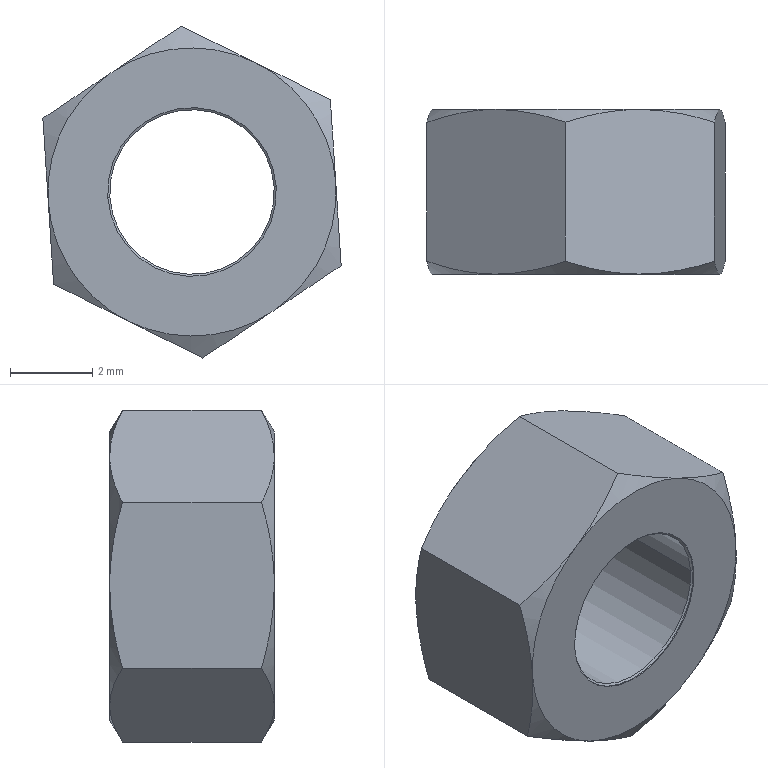Component | SolidWorks | hex nut style 2_am_pkg-24 | 1 solid | 28 faces | box 7.25 x 4 x 8.07 mm | volume 119 mm3 | cone 16 | plane 8 | cylinder 4 | commonest cylinder face diameters 4.1 x2 4 x2
STEP:
#1=COLOUR_RGB('',0.7922,0.8196,0.9333);
#2=FILL_AREA_STYLE_COLOUR('',#1);
#3=FILL_AREA_STYLE('',(#2));
#4=SURFACE_STYLE_FILL_AREA(#3);
#5=SURFACE_SIDE_STYLE('',(#4));
#6=SURFACE_STYLE_USAGE(.BOTH.,#5);
#7=PRESENTATION_STYLE_ASSIGNMENT((#6));
#8=CARTESIAN_POINT('',(-3.26,1.437,3.346));
#9=VERTEX_POINT('',#8);
#10=CARTESIAN_POINT('',(-3.421,1.437,3.335));
#11=VERTEX_POINT('',#10);
#12=CARTESIAN_POINT('',(-3.341,1.437,3.341));
#13=DIRECTION('',(-0.,1.,0.));
#14=DIRECTION('',(0.9979,0.,0.06475));
#15=AXIS2_PLACEMENT_3D('',#12,#13,#14);
#16=CIRCLE('',#15,0.08071);
#17=EDGE_CURVE('',#9,#11,#16,.T.);
#18=ORIENTED_EDGE('',*,*,#17,.F.);
#19=CARTESIAN_POINT('',(-3.26,1.438,3.346));
#20=VERTEX_POINT('',#19);
#21=CARTESIAN_POINT('',(-3.26,0.6088,3.346));
#22=DIRECTION('',(-0.,1.,0.));
#23=VECTOR('',#22,39.37);
#24=LINE('',#21,#23);
#25=EDGE_CURVE('',#9,#20,#24,.T.);
#26=ORIENTED_EDGE('',*,*,#25,.T.);
#27=CARTESIAN_POINT('',(-3.421,1.438,3.335));
#28=VERTEX_POINT('',#27);
#29=CARTESIAN_POINT('',(-3.341,1.438,3.341));
#30=DIRECTION('',(-0.,1.,0.));
#31=DIRECTION('',(-0.9979,0.,-0.06475));
#32=AXIS2_PLACEMENT_3D('',#29,#30,#31);
#33=CIRCLE('',#32,0.08071);
#34=EDGE_CURVE('',#20,#28,#33,.T.);
#35=ORIENTED_EDGE('',*,*,#34,.T.);
#36=CARTESIAN_POINT('',(-3.421,0.6088,3.335));
#37=DIRECTION('',(-0.,1.,0.));
#38=VECTOR('',#37,39.37);
#39=LINE('',#36,#38);
#40=EDGE_CURVE('',#11,#28,#39,.T.);
#41=ORIENTED_EDGE('',*,*,#40,.F.);
#42=EDGE_LOOP('',(#18,#26,#35,#41));
#43=FACE_OUTER_BOUND('',#42,.T.);
#44=CARTESIAN_POINT('',(-3.341,0.6088,3.341));
#45=DIRECTION('',(-0.,1.,0.));
#46=DIRECTION('',(-0.9979,0.,-0.06475));
#47=AXIS2_PLACEMENT_3D('',#44,#45,#46);
#48=CYLINDRICAL_SURFACE('',#47,0.08071);
#49=ADVANCED_FACE('',(#43),#48,.F.);
#50=CARTESIAN_POINT('',(-3.262,1.439,3.346));
#51=VERTEX_POINT('',#50);
#52=CARTESIAN_POINT('',(-3.419,1.439,3.336));
#53=VERTEX_POINT('',#52);
#54=CARTESIAN_POINT('',(-3.341,1.439,3.341));
#55=DIRECTION('',(-0.,1.,0.));
#56=DIRECTION('',(0.9979,0.,0.06475));
#57=AXIS2_PLACEMENT_3D('',#54,#55,#56);
#58=CIRCLE('',#57,0.07874);
#59=EDGE_CURVE('',#51,#53,#58,.T.);
#60=ORIENTED_EDGE('',*,*,#59,.T.);
#61=CARTESIAN_POINT('',(-3.421,1.438,3.335));
#62=DIRECTION('',(-0.8174,-0.5736,-0.05304));
#63=VECTOR('',#62,39.37);
#64=LINE('',#61,#63);
#65=EDGE_CURVE('',#53,#28,#64,.T.);
#66=ORIENTED_EDGE('',*,*,#65,.T.);
#67=ORIENTED_EDGE('',*,*,#34,.F.);
#68=CARTESIAN_POINT('',(-3.26,1.438,3.346));
#69=DIRECTION('',(0.8174,-0.5736,0.05304));
#70=VECTOR('',#69,39.37);
#71=LINE('',#68,#70);
#72=EDGE_CURVE('',#51,#20,#71,.T.);
#73=ORIENTED_EDGE('',*,*,#72,.F.);
#74=EDGE_LOOP('',(#60,#66,#67,#73));
#75=FACE_OUTER_BOUND('',#74,.T.);
#76=CARTESIAN_POINT('',(-3.341,1.438,3.341));
#77=DIRECTION('',(0.,-1.,-0.));
#78=DIRECTION('',(0.9979,0.,0.06475));
#79=AXIS2_PLACEMENT_3D('',#76,#77,#78);
#80=CONICAL_SURFACE('',#79,0.08071,0.9599);
#81=ADVANCED_FACE('',(#75),#80,.F.);
#82=CARTESIAN_POINT('',(-3.419,1.593,3.336));
#83=VERTEX_POINT('',#82);
#84=CARTESIAN_POINT('',(-3.262,1.593,3.346));
#85=VERTEX_POINT('',#84);
#86=CARTESIAN_POINT('',(-3.341,1.593,3.341));
#87=DIRECTION('',(0.,-1.,-0.));
#88=DIRECTION('',(-0.9979,0.,-0.06475));
#89=AXIS2_PLACEMENT_3D('',#86,#87,#88);
#90=CIRCLE('',#89,0.07874);
#91=EDGE_CURVE('',#83,#85,#90,.T.);
#92=ORIENTED_EDGE('',*,*,#91,.T.);
#93=CARTESIAN_POINT('',(-3.26,1.594,3.346));
#94=VERTEX_POINT('',#93);
#95=CARTESIAN_POINT('',(-3.262,1.593,3.346));
#96=DIRECTION('',(0.8174,0.5736,0.05304));
#97=VECTOR('',#96,39.37);
#98=LINE('',#95,#97);
#99=EDGE_CURVE('',#85,#94,#98,.T.);
#100=ORIENTED_EDGE('',*,*,#99,.T.);
#101=CARTESIAN_POINT('',(-3.421,1.594,3.335));
#102=VERTEX_POINT('',#101);
#103=CARTESIAN_POINT('',(-3.341,1.594,3.341));
#104=DIRECTION('',(-0.,1.,0.));
#105=DIRECTION('',(-0.9979,0.,-0.06475));
#106=AXIS2_PLACEMENT_3D('',#103,#104,#105);
#107=CIRCLE('',#106,0.08071);
#108=EDGE_CURVE('',#94,#102,#107,.T.);
#109=ORIENTED_EDGE('',*,*,#108,.T.);
#110=CARTESIAN_POINT('',(-3.419,1.593,3.336));
#111=DIRECTION('',(-0.8174,0.5736,-0.05304));
#112=VECTOR('',#111,39.37);
#113=LINE('',#110,#112);
#114=EDGE_CURVE('',#83,#102,#113,.T.);
#115=ORIENTED_EDGE('',*,*,#114,.F.);
#116=EDGE_LOOP('',(#92,#100,#109,#115));
#117=FACE_OUTER_BOUND('',#116,.T.);
#118=CARTESIAN_POINT('',(-3.341,1.593,3.341));
#119=DIRECTION('',(-0.,1.,0.));
#120=DIRECTION('',(-0.9979,0.,-0.06475));
#121=AXIS2_PLACEMENT_3D('',#118,#119,#120);
#122=CONICAL_SURFACE('',#121,0.07854,0.9599);
#123=ADVANCED_FACE('',(#117),#122,.F.);
#124=ORIENTED_EDGE('',*,*,#59,.F.);
#125=CARTESIAN_POINT('',(-3.262,1.437,3.346));
#126=DIRECTION('',(-0.,1.,0.));
#127=VECTOR('',#126,39.37);
#128=LINE('',#125,#127);
#129=EDGE_CURVE('',#51,#85,#128,.T.);
#130=ORIENTED_EDGE('',*,*,#129,.T.);
#131=ORIENTED_EDGE('',*,*,#91,.F.);
#132=CARTESIAN_POINT('',(-3.419,1.437,3.336));
#133=DIRECTION('',(-0.,1.,0.));
#134=VECTOR('',#133,39.37);
#135=LINE('',#132,#134);
#136=EDGE_CURVE('',#53,#83,#135,.T.);
#137=ORIENTED_EDGE('',*,*,#136,.F.);
#138=EDGE_LOOP('',(#124,#130,#131,#137));
#139=FACE_OUTER_BOUND('',#138,.T.);
#140=CARTESIAN_POINT('',(-3.341,1.437,3.341));
#141=DIRECTION('',(-0.,1.,0.));
#142=DIRECTION('',(-0.9979,0.,-0.06475));
#143=AXIS2_PLACEMENT_3D('',#140,#141,#142);
#144=CYLINDRICAL_SURFACE('',#143,0.07874);
#145=ADVANCED_FACE('',(#139),#144,.F.);
#146=ORIENTED_EDGE('',*,*,#129,.F.);
#147=CARTESIAN_POINT('',(-3.341,1.439,3.341));
#148=DIRECTION('',(-0.,1.,0.));
#149=DIRECTION('',(0.9979,0.,0.06475));
#150=AXIS2_PLACEMENT_3D('',#147,#148,#149);
#151=CIRCLE('',#150,0.07874);
#152=EDGE_CURVE('',#53,#51,#151,.T.);
#153=ORIENTED_EDGE('',*,*,#152,.F.);
#154=ORIENTED_EDGE('',*,*,#136,.T.);
#155=CARTESIAN_POINT('',(-3.341,1.593,3.341));
#156=DIRECTION('',(0.,-1.,-0.));
#157=DIRECTION('',(-0.9979,0.,-0.06475));
#158=AXIS2_PLACEMENT_3D('',#155,#156,#157);
#159=CIRCLE('',#158,0.07874);
#160=EDGE_CURVE('',#85,#83,#159,.T.);
#161=ORIENTED_EDGE('',*,*,#160,.F.);
#162=EDGE_LOOP('',(#146,#153,#154,#161));
#163=FACE_OUTER_BOUND('',#162,.T.);
#164=CARTESIAN_POINT('',(-3.341,1.437,3.341));
#165=DIRECTION('',(-0.,1.,0.));
#166=DIRECTION('',(-0.9979,0.,-0.06475));
#167=AXIS2_PLACEMENT_3D('',#164,#165,#166);
#168=CYLINDRICAL_SURFACE('',#167,0.07874);
#169=ADVANCED_FACE('',(#163),#168,.F.);
#170=CARTESIAN_POINT('',(-3.208,1.449,3.429));
#171=VERTEX_POINT('',#170);
#172=CARTESIAN_POINT('',(-3.208,1.582,3.429));
#173=VERTEX_POINT('',#172);
#174=CARTESIAN_POINT('',(-3.208,1.437,3.429));
#175=DIRECTION('',(-0.,1.,0.));
#176=VECTOR('',#175,39.37);
#177=LINE('',#174,#176);
#178=EDGE_CURVE('',#171,#173,#177,.T.);
#179=ORIENTED_EDGE('',*,*,#178,.T.);
#180=CARTESIAN_POINT('',(-3.28,1.594,3.464));
#181=VERTEX_POINT('',#180);
#182=CARTESIAN_POINT('',(-3.208,1.582,3.429));
#183=CARTESIAN_POINT('',(-3.232,1.59,3.441));
#184=CARTESIAN_POINT('',(-3.255,1.594,3.452));
#185=CARTESIAN_POINT('',(-3.28,1.594,3.464));
#186=B_SPLINE_CURVE_WITH_KNOTS('',3,(#182,#183,#184,#185),.UNSPECIFIED.,.F.,.F.,(4,4),(0.00000024,0.002045),.UNSPECIFIED.);
#187=EDGE_CURVE('',#173,#181,#186,.T.);
#188=ORIENTED_EDGE('',*,*,#187,.T.);
#189=CARTESIAN_POINT('',(-3.351,1.582,3.499));
#190=VERTEX_POINT('',#189);
#191=CARTESIAN_POINT('',(-3.28,1.594,3.464));
#192=CARTESIAN_POINT('',(-3.292,1.594,3.47));
#193=CARTESIAN_POINT('',(-3.304,1.593,3.476));
#194=CARTESIAN_POINT('',(-3.328,1.589,3.488));
#195=CARTESIAN_POINT('',(-3.339,1.586,3.494));
#196=CARTESIAN_POINT('',(-3.351,1.582,3.499));
#197=B_SPLINE_CURVE_WITH_KNOTS('',3,(#191,#192,#193,#194,#195,#196),.UNSPECIFIED.,.F.,.F.,(4,2,4),(0.002045,0.003063,0.004082),.UNSPECIFIED.);
#198=EDGE_CURVE('',#181,#190,#197,.T.);
#199=ORIENTED_EDGE('',*,*,#198,.T.);
#200=CARTESIAN_POINT('',(-3.351,1.449,3.499));
#201=VERTEX_POINT('',#200);
#202=CARTESIAN_POINT('',(-3.351,1.437,3.499));
#203=DIRECTION('',(-0.,1.,0.));
#204=VECTOR('',#203,39.37);
#205=LINE('',#202,#204);
#206=EDGE_CURVE('',#201,#190,#205,.T.);
#207=ORIENTED_EDGE('',*,*,#206,.F.);
#208=CARTESIAN_POINT('',(-3.28,1.437,3.464));
#209=VERTEX_POINT('',#208);
#210=CARTESIAN_POINT('',(-3.28,1.437,3.464));
#211=CARTESIAN_POINT('',(-3.292,1.437,3.47));
#212=CARTESIAN_POINT('',(-3.304,1.438,3.476));
#213=CARTESIAN_POINT('',(-3.328,1.442,3.488));
#214=CARTESIAN_POINT('',(-3.339,1.446,3.494));
#215=CARTESIAN_POINT('',(-3.351,1.449,3.499));
#216=B_SPLINE_CURVE_WITH_KNOTS('',3,(#210,#211,#212,#213,#214,#215),.UNSPECIFIED.,.F.,.F.,(4,2,4),(0.002045,0.003063,0.004082),.UNSPECIFIED.);
#217=EDGE_CURVE('',#209,#201,#216,.T.);
#218=ORIENTED_EDGE('',*,*,#217,.F.);
#219=CARTESIAN_POINT('',(-3.208,1.449,3.429));
#220=CARTESIAN_POINT('',(-3.232,1.442,3.441));
#221=CARTESIAN_POINT('',(-3.255,1.437,3.452));
#222=CARTESIAN_POINT('',(-3.28,1.437,3.464));
#223=B_SPLINE_CURVE_WITH_KNOTS('',3,(#219,#220,#221,#222),.UNSPECIFIED.,.F.,.F.,(4,4),(0.00000024,0.002045),.UNSPECIFIED.);
#224=EDGE_CURVE('',#171,#209,#223,.T.);
#225=ORIENTED_EDGE('',*,*,#224,.F.);
#226=EDGE_LOOP('',(#179,#188,#199,#207,#218,#225));
#227=FACE_OUTER_BOUND('',#226,.T.);
#228=CARTESIAN_POINT('',(-3.351,1.437,3.499));
#229=DIRECTION('',(0.4429,0.,0.8966));
#230=DIRECTION('',(0.8966,0.,-0.4429));
#231=AXIS2_PLACEMENT_3D('',#228,#229,#230);
#232=PLANE('',#231);
#233=ADVANCED_FACE('',(#227),#232,.T.);
#234=ORIENTED_EDGE('',*,*,#206,.T.);
#235=CARTESIAN_POINT('',(-3.417,1.594,3.455));
#236=VERTEX_POINT('',#235);
#237=CARTESIAN_POINT('',(-3.351,1.582,3.499));
#238=CARTESIAN_POINT('',(-3.373,1.59,3.485));
#239=CARTESIAN_POINT('',(-3.395,1.594,3.47));
#240=CARTESIAN_POINT('',(-3.417,1.594,3.455));
#241=B_SPLINE_CURVE_WITH_KNOTS('',3,(#237,#238,#239,#240),.UNSPECIFIED.,.F.,.F.,(4,4),(0.00000024,0.002045),.UNSPECIFIED.);
#242=EDGE_CURVE('',#190,#236,#241,.T.);
#243=ORIENTED_EDGE('',*,*,#242,.T.);
#244=CARTESIAN_POINT('',(-3.483,1.582,3.411));
#245=VERTEX_POINT('',#244);
#246=CARTESIAN_POINT('',(-3.417,1.594,3.455));
#247=CARTESIAN_POINT('',(-3.428,1.594,3.448));
#248=CARTESIAN_POINT('',(-3.44,1.593,3.44));
#249=CARTESIAN_POINT('',(-3.462,1.589,3.426));
#250=CARTESIAN_POINT('',(-3.473,1.586,3.418));
#251=CARTESIAN_POINT('',(-3.483,1.582,3.411));
#252=B_SPLINE_CURVE_WITH_KNOTS('',3,(#246,#247,#248,#249,#250,#251),.UNSPECIFIED.,.F.,.F.,(4,2,4),(0.002045,0.003063,0.004082),.UNSPECIFIED.);
#253=EDGE_CURVE('',#236,#245,#252,.T.);
#254=ORIENTED_EDGE('',*,*,#253,.T.);
#255=CARTESIAN_POINT('',(-3.483,1.449,3.411));
#256=VERTEX_POINT('',#255);
#257=CARTESIAN_POINT('',(-3.483,1.437,3.411));
#258=DIRECTION('',(-0.,1.,0.));
#259=VECTOR('',#258,39.37);
#260=LINE('',#257,#259);
#261=EDGE_CURVE('',#256,#245,#260,.T.);
#262=ORIENTED_EDGE('',*,*,#261,.F.);
#263=CARTESIAN_POINT('',(-3.417,1.437,3.455));
#264=VERTEX_POINT('',#263);
#265=CARTESIAN_POINT('',(-3.417,1.437,3.455));
#266=CARTESIAN_POINT('',(-3.428,1.437,3.448));
#267=CARTESIAN_POINT('',(-3.44,1.438,3.44));
#268=CARTESIAN_POINT('',(-3.462,1.442,3.426));
#269=CARTESIAN_POINT('',(-3.473,1.446,3.418));
#270=CARTESIAN_POINT('',(-3.483,1.449,3.411));
#271=B_SPLINE_CURVE_WITH_KNOTS('',3,(#265,#266,#267,#268,#269,#270),.UNSPECIFIED.,.F.,.F.,(4,2,4),(0.002045,0.003063,0.004082),.UNSPECIFIED.);
#272=EDGE_CURVE('',#264,#256,#271,.T.);
#273=ORIENTED_EDGE('',*,*,#272,.F.);
#274=CARTESIAN_POINT('',(-3.351,1.449,3.499));
#275=CARTESIAN_POINT('',(-3.373,1.442,3.485));
#276=CARTESIAN_POINT('',(-3.395,1.437,3.47));
#277=CARTESIAN_POINT('',(-3.417,1.437,3.455));
#278=B_SPLINE_CURVE_WITH_KNOTS('',3,(#274,#275,#276,#277),.UNSPECIFIED.,.F.,.F.,(4,4),(0.00000024,0.002045),.UNSPECIFIED.);
#279=EDGE_CURVE('',#201,#264,#278,.T.);
#280=ORIENTED_EDGE('',*,*,#279,.F.);
#281=EDGE_LOOP('',(#234,#243,#254,#262,#273,#280));
#282=FACE_OUTER_BOUND('',#281,.T.);
#283=CARTESIAN_POINT('',(-3.483,1.437,3.411));
#284=DIRECTION('',(-0.555,-0.,0.8318));
#285=DIRECTION('',(0.8318,0.,0.555));
#286=AXIS2_PLACEMENT_3D('',#283,#284,#285);
#287=PLANE('',#286);
#288=ADVANCED_FACE('',(#282),#287,.T.);
#289=CARTESIAN_POINT('',(-3.473,1.582,3.252));
#290=VERTEX_POINT('',#289);
#291=CARTESIAN_POINT('',(-3.478,1.594,3.332));
#292=VERTEX_POINT('',#291);
#293=CARTESIAN_POINT('',(-3.473,1.582,3.252));
#294=CARTESIAN_POINT('',(-3.474,1.586,3.265));
#295=CARTESIAN_POINT('',(-3.475,1.589,3.278));
#296=CARTESIAN_POINT('',(-3.476,1.593,3.305));
#297=CARTESIAN_POINT('',(-3.477,1.594,3.318));
#298=CARTESIAN_POINT('',(-3.478,1.594,3.332));
#299=B_SPLINE_CURVE_WITH_KNOTS('',3,(#293,#294,#295,#296,#297,#298),.UNSPECIFIED.,.F.,.F.,(4,2,4),(0.003605,0.004627,0.005649),.UNSPECIFIED.);
#300=EDGE_CURVE('',#290,#292,#299,.T.);
#301=ORIENTED_EDGE('',*,*,#300,.F.);
#302=CARTESIAN_POINT('',(-3.473,1.449,3.252));
#303=VERTEX_POINT('',#302);
#304=CARTESIAN_POINT('',(-3.473,1.437,3.252));
#305=DIRECTION('',(-0.,1.,0.));
#306=VECTOR('',#305,39.37);
#307=LINE('',#304,#306);
#308=EDGE_CURVE('',#303,#290,#307,.T.);
#309=ORIENTED_EDGE('',*,*,#308,.F.);
#310=CARTESIAN_POINT('',(-3.478,1.437,3.332));
#311=VERTEX_POINT('',#310);
#312=CARTESIAN_POINT('',(-3.473,1.449,3.252));
#313=CARTESIAN_POINT('',(-3.474,1.446,3.265));
#314=CARTESIAN_POINT('',(-3.475,1.442,3.278));
#315=CARTESIAN_POINT('',(-3.476,1.438,3.305));
#316=CARTESIAN_POINT('',(-3.477,1.437,3.318));
#317=CARTESIAN_POINT('',(-3.478,1.437,3.332));
#318=B_SPLINE_CURVE_WITH_KNOTS('',3,(#312,#313,#314,#315,#316,#317),.UNSPECIFIED.,.F.,.F.,(4,2,4),(0.003605,0.004627,0.005649),.UNSPECIFIED.);
#319=EDGE_CURVE('',#303,#311,#318,.T.);
#320=ORIENTED_EDGE('',*,*,#319,.T.);
#321=CARTESIAN_POINT('',(-3.478,1.437,3.332));
#322=CARTESIAN_POINT('',(-3.479,1.437,3.345));
#323=CARTESIAN_POINT('',(-3.48,1.438,3.359));
#324=CARTESIAN_POINT('',(-3.482,1.443,3.385));
#325=CARTESIAN_POINT('',(-3.482,1.446,3.398));
#326=CARTESIAN_POINT('',(-3.483,1.449,3.411));
#327=B_SPLINE_CURVE_WITH_KNOTS('',3,(#321,#322,#323,#324,#325,#326),.UNSPECIFIED.,.F.,.F.,(4,2,4),(0.005649,0.006672,0.007695),.UNSPECIFIED.);
#328=EDGE_CURVE('',#311,#256,#327,.T.);
#329=ORIENTED_EDGE('',*,*,#328,.T.);
#330=ORIENTED_EDGE('',*,*,#261,.T.);
#331=CARTESIAN_POINT('',(-3.478,1.594,3.332));
#332=CARTESIAN_POINT('',(-3.479,1.594,3.345));
#333=CARTESIAN_POINT('',(-3.48,1.593,3.359));
#334=CARTESIAN_POINT('',(-3.482,1.589,3.385));
#335=CARTESIAN_POINT('',(-3.482,1.586,3.398));
#336=CARTESIAN_POINT('',(-3.483,1.582,3.411));
#337=B_SPLINE_CURVE_WITH_KNOTS('',3,(#331,#332,#333,#334,#335,#336),.UNSPECIFIED.,.F.,.F.,(4,2,4),(0.005649,0.006672,0.007695),.UNSPECIFIED.);
#338=EDGE_CURVE('',#292,#245,#337,.T.);
#339=ORIENTED_EDGE('',*,*,#338,.F.);
#340=EDGE_LOOP('',(#301,#309,#320,#329,#330,#339));
#341=FACE_OUTER_BOUND('',#340,.T.);
#342=CARTESIAN_POINT('',(-3.483,1.437,3.411));
#343=DIRECTION('',(0.9979,0.,0.06475));
#344=DIRECTION('',(-0.,1.,0.));
#345=AXIS2_PLACEMENT_3D('',#342,#343,#344);
#346=PLANE('',#345);
#347=ADVANCED_FACE('',(#341),#346,.F.);
#348=ORIENTED_EDGE('',*,*,#308,.T.);
#349=CARTESIAN_POINT('',(-3.402,1.594,3.217));
#350=VERTEX_POINT('',#349);
#351=CARTESIAN_POINT('',(-3.473,1.582,3.252));
#352=CARTESIAN_POINT('',(-3.45,1.59,3.241));
#353=CARTESIAN_POINT('',(-3.426,1.594,3.229));
#354=CARTESIAN_POINT('',(-3.402,1.594,3.217));
#355=B_SPLINE_CURVE_WITH_KNOTS('',3,(#351,#352,#353,#354),.UNSPECIFIED.,.F.,.F.,(4,4),(0.00000024,0.002045),.UNSPECIFIED.);
#356=EDGE_CURVE('',#290,#350,#355,.T.);
#357=ORIENTED_EDGE('',*,*,#356,.T.);
#358=CARTESIAN_POINT('',(-3.33,1.582,3.182));
#359=VERTEX_POINT('',#358);
#360=CARTESIAN_POINT('',(-3.402,1.594,3.217));
#361=CARTESIAN_POINT('',(-3.39,1.594,3.211));
#362=CARTESIAN_POINT('',(-3.377,1.593,3.205));
#363=CARTESIAN_POINT('',(-3.354,1.589,3.193));
#364=CARTESIAN_POINT('',(-3.342,1.586,3.188));
#365=CARTESIAN_POINT('',(-3.33,1.582,3.182));
#366=B_SPLINE_CURVE_WITH_KNOTS('',3,(#360,#361,#362,#363,#364,#365),.UNSPECIFIED.,.F.,.F.,(4,2,4),(0.002045,0.003063,0.004082),.UNSPECIFIED.);
#367=EDGE_CURVE('',#350,#359,#366,.T.);
#368=ORIENTED_EDGE('',*,*,#367,.T.);
#369=CARTESIAN_POINT('',(-3.33,1.449,3.182));
#370=VERTEX_POINT('',#369);
#371=CARTESIAN_POINT('',(-3.33,1.437,3.182));
#372=DIRECTION('',(-0.,1.,0.));
#373=VECTOR('',#372,39.37);
#374=LINE('',#371,#373);
#375=EDGE_CURVE('',#370,#359,#374,.T.);
#376=ORIENTED_EDGE('',*,*,#375,.F.);
#377=CARTESIAN_POINT('',(-3.402,1.437,3.217));
#378=VERTEX_POINT('',#377);
#379=CARTESIAN_POINT('',(-3.402,1.437,3.217));
#380=CARTESIAN_POINT('',(-3.39,1.437,3.211));
#381=CARTESIAN_POINT('',(-3.377,1.438,3.205));
#382=CARTESIAN_POINT('',(-3.354,1.442,3.193));
#383=CARTESIAN_POINT('',(-3.342,1.446,3.188));
#384=CARTESIAN_POINT('',(-3.33,1.449,3.182));
#385=B_SPLINE_CURVE_WITH_KNOTS('',3,(#379,#380,#381,#382,#383,#384),.UNSPECIFIED.,.F.,.F.,(4,2,4),(0.002045,0.003063,0.004082),.UNSPECIFIED.);
#386=EDGE_CURVE('',#378,#370,#385,.T.);
#387=ORIENTED_EDGE('',*,*,#386,.F.);
#388=CARTESIAN_POINT('',(-3.473,1.449,3.252));
#389=CARTESIAN_POINT('',(-3.45,1.442,3.241));
#390=CARTESIAN_POINT('',(-3.426,1.437,3.229));
#391=CARTESIAN_POINT('',(-3.402,1.437,3.217));
#392=B_SPLINE_CURVE_WITH_KNOTS('',3,(#388,#389,#390,#391),.UNSPECIFIED.,.F.,.F.,(4,4),(0.00000024,0.002045),.UNSPECIFIED.);
#393=EDGE_CURVE('',#303,#378,#392,.T.);
#394=ORIENTED_EDGE('',*,*,#393,.F.);
#395=EDGE_LOOP('',(#348,#357,#368,#376,#387,#394));
#396=FACE_OUTER_BOUND('',#395,.T.);
#397=CARTESIAN_POINT('',(-3.33,1.437,3.182));
#398=DIRECTION('',(-0.4429,-0.,-0.8966));
#399=DIRECTION('',(-0.8966,-0.,0.4429));
#400=AXIS2_PLACEMENT_3D('',#397,#398,#399);
#401=PLANE('',#400);
#402=ADVANCED_FACE('',(#396),#401,.T.);
#403=ORIENTED_EDGE('',*,*,#375,.T.);
#404=CARTESIAN_POINT('',(-3.264,1.594,3.226));
#405=VERTEX_POINT('',#404);
#406=CARTESIAN_POINT('',(-3.33,1.582,3.182));
#407=CARTESIAN_POINT('',(-3.309,1.59,3.196));
#408=CARTESIAN_POINT('',(-3.287,1.594,3.211));
#409=CARTESIAN_POINT('',(-3.264,1.594,3.226));
#410=B_SPLINE_CURVE_WITH_KNOTS('',3,(#406,#407,#408,#409),.UNSPECIFIED.,.F.,.F.,(4,4),(0.00000024,0.002045),.UNSPECIFIED.);
#411=EDGE_CURVE('',#359,#405,#410,.T.);
#412=ORIENTED_EDGE('',*,*,#411,.T.);
#413=CARTESIAN_POINT('',(-3.198,1.582,3.27));
#414=VERTEX_POINT('',#413);
#415=CARTESIAN_POINT('',(-3.264,1.594,3.226));
#416=CARTESIAN_POINT('',(-3.253,1.594,3.234));
#417=CARTESIAN_POINT('',(-3.242,1.593,3.241));
#418=CARTESIAN_POINT('',(-3.22,1.589,3.256));
#419=CARTESIAN_POINT('',(-3.209,1.586,3.263));
#420=CARTESIAN_POINT('',(-3.198,1.582,3.27));
#421=B_SPLINE_CURVE_WITH_KNOTS('',3,(#415,#416,#417,#418,#419,#420),.UNSPECIFIED.,.F.,.F.,(4,2,4),(0.002045,0.003063,0.004082),.UNSPECIFIED.);
#422=EDGE_CURVE('',#405,#414,#421,.T.);
#423=ORIENTED_EDGE('',*,*,#422,.T.);
#424=CARTESIAN_POINT('',(-3.198,1.449,3.27));
#425=VERTEX_POINT('',#424);
#426=CARTESIAN_POINT('',(-3.198,1.437,3.27));
#427=DIRECTION('',(-0.,1.,0.));
#428=VECTOR('',#427,39.37);
#429=LINE('',#426,#428);
#430=EDGE_CURVE('',#425,#414,#429,.T.);
#431=ORIENTED_EDGE('',*,*,#430,.F.);
#432=CARTESIAN_POINT('',(-3.264,1.437,3.226));
#433=VERTEX_POINT('',#432);
#434=CARTESIAN_POINT('',(-3.264,1.437,3.226));
#435=CARTESIAN_POINT('',(-3.253,1.437,3.234));
#436=CARTESIAN_POINT('',(-3.242,1.438,3.241));
#437=CARTESIAN_POINT('',(-3.22,1.442,3.256));
#438=CARTESIAN_POINT('',(-3.209,1.446,3.263));
#439=CARTESIAN_POINT('',(-3.198,1.449,3.27));
#440=B_SPLINE_CURVE_WITH_KNOTS('',3,(#434,#435,#436,#437,#438,#439),.UNSPECIFIED.,.F.,.F.,(4,2,4),(0.002045,0.003063,0.004082),.UNSPECIFIED.);
#441=EDGE_CURVE('',#433,#425,#440,.T.);
#442=ORIENTED_EDGE('',*,*,#441,.F.);
#443=CARTESIAN_POINT('',(-3.33,1.449,3.182));
#444=CARTESIAN_POINT('',(-3.309,1.442,3.196));
#445=CARTESIAN_POINT('',(-3.287,1.437,3.211));
#446=CARTESIAN_POINT('',(-3.264,1.437,3.226));
#447=B_SPLINE_CURVE_WITH_KNOTS('',3,(#443,#444,#445,#446),.UNSPECIFIED.,.F.,.F.,(4,4),(0.00000024,0.002045),.UNSPECIFIED.);
#448=EDGE_CURVE('',#370,#433,#447,.T.);
#449=ORIENTED_EDGE('',*,*,#448,.F.);
#450=EDGE_LOOP('',(#403,#412,#423,#431,#442,#449));
#451=FACE_OUTER_BOUND('',#450,.T.);
#452=CARTESIAN_POINT('',(-3.198,1.437,3.27));
#453=DIRECTION('',(0.555,0.,-0.8318));
#454=DIRECTION('',(-0.8318,-0.,-0.555));
#455=AXIS2_PLACEMENT_3D('',#452,#453,#454);
#456=PLANE('',#455);
#457=ADVANCED_FACE('',(#451),#456,.T.);
#458=ORIENTED_EDGE('',*,*,#430,.T.);
#459=CARTESIAN_POINT('',(-3.203,1.594,3.35));
#460=VERTEX_POINT('',#459);
#461=CARTESIAN_POINT('',(-3.198,1.582,3.27));
#462=CARTESIAN_POINT('',(-3.199,1.586,3.283));
#463=CARTESIAN_POINT('',(-3.2,1.589,3.296));
#464=CARTESIAN_POINT('',(-3.201,1.593,3.323));
#465=CARTESIAN_POINT('',(-3.202,1.594,3.336));
#466=CARTESIAN_POINT('',(-3.203,1.594,3.35));
#467=B_SPLINE_CURVE_WITH_KNOTS('',3,(#461,#462,#463,#464,#465,#466),.UNSPECIFIED.,.F.,.F.,(4,2,4),(0.003605,0.004627,0.005649),.UNSPECIFIED.);
#468=EDGE_CURVE('',#414,#460,#467,.T.);
#469=ORIENTED_EDGE('',*,*,#468,.T.);
#470=CARTESIAN_POINT('',(-3.203,1.594,3.35));
#471=CARTESIAN_POINT('',(-3.204,1.594,3.363));
#472=CARTESIAN_POINT('',(-3.205,1.593,3.377));
#473=CARTESIAN_POINT('',(-3.207,1.589,3.403));
#474=CARTESIAN_POINT('',(-3.207,1.586,3.416));
#475=CARTESIAN_POINT('',(-3.208,1.582,3.429));
#476=B_SPLINE_CURVE_WITH_KNOTS('',3,(#470,#471,#472,#473,#474,#475),.UNSPECIFIED.,.F.,.F.,(4,2,4),(0.005649,0.006672,0.007695),.UNSPECIFIED.);
#477=EDGE_CURVE('',#460,#173,#476,.T.);
#478=ORIENTED_EDGE('',*,*,#477,.T.);
#479=ORIENTED_EDGE('',*,*,#178,.F.);
#480=CARTESIAN_POINT('',(-3.203,1.437,3.35));
#481=VERTEX_POINT('',#480);
#482=CARTESIAN_POINT('',(-3.203,1.437,3.35));
#483=CARTESIAN_POINT('',(-3.204,1.437,3.363));
#484=CARTESIAN_POINT('',(-3.205,1.438,3.377));
#485=CARTESIAN_POINT('',(-3.207,1.443,3.403));
#486=CARTESIAN_POINT('',(-3.207,1.446,3.416));
#487=CARTESIAN_POINT('',(-3.208,1.449,3.429));
#488=B_SPLINE_CURVE_WITH_KNOTS('',3,(#482,#483,#484,#485,#486,#487),.UNSPECIFIED.,.F.,.F.,(4,2,4),(0.005649,0.006672,0.007695),.UNSPECIFIED.);
#489=EDGE_CURVE('',#481,#171,#488,.T.);
#490=ORIENTED_EDGE('',*,*,#489,.F.);
#491=CARTESIAN_POINT('',(-3.198,1.449,3.27));
#492=CARTESIAN_POINT('',(-3.199,1.446,3.283));
#493=CARTESIAN_POINT('',(-3.2,1.442,3.296));
#494=CARTESIAN_POINT('',(-3.201,1.438,3.323));
#495=CARTESIAN_POINT('',(-3.202,1.437,3.336));
#496=CARTESIAN_POINT('',(-3.203,1.437,3.35));
#497=B_SPLINE_CURVE_WITH_KNOTS('',3,(#491,#492,#493,#494,#495,#496),.UNSPECIFIED.,.F.,.F.,(4,2,4),(0.003605,0.004627,0.005649),.UNSPECIFIED.);
#498=EDGE_CURVE('',#425,#481,#497,.T.);
#499=ORIENTED_EDGE('',*,*,#498,.F.);
#500=EDGE_LOOP('',(#458,#469,#478,#479,#490,#499));
#501=FACE_OUTER_BOUND('',#500,.T.);
#502=CARTESIAN_POINT('',(-3.208,1.437,3.429));
#503=DIRECTION('',(0.9979,0.,0.06475));
#504=DIRECTION('',(-0.,1.,0.));
#505=AXIS2_PLACEMENT_3D('',#502,#503,#504);
#506=PLANE('',#505);
#507=ADVANCED_FACE('',(#501),#506,.T.);
#508=CARTESIAN_POINT('',(-3.341,1.594,3.341));
#509=DIRECTION('',(-0.,1.,0.));
#510=DIRECTION('',(-0.9979,0.,-0.06475));
#511=AXIS2_PLACEMENT_3D('',#508,#509,#510);
#512=CIRCLE('',#511,0.08071);
#513=EDGE_CURVE('',#102,#94,#512,.T.);
#514=ORIENTED_EDGE('',*,*,#513,.F.);
#515=ORIENTED_EDGE('',*,*,#108,.F.);
#516=EDGE_LOOP('',(#514,#515));
#517=FACE_BOUND('',#516,.T.);
#518=CARTESIAN_POINT('',(-3.341,1.594,3.341));
#519=DIRECTION('',(0.,-1.,-0.));
#520=DIRECTION('',(0.9979,0.,0.06475));
#521=AXIS2_PLACEMENT_3D('',#518,#519,#520);
#522=CIRCLE('',#521,0.1378);
#523=EDGE_CURVE('',#460,#181,#522,.T.);
#524=ORIENTED_EDGE('',*,*,#523,.F.);
#525=CARTESIAN_POINT('',(-3.341,1.594,3.341));
#526=DIRECTION('',(0.,-1.,-0.));
#527=DIRECTION('',(0.9979,0.,0.06475));
#528=AXIS2_PLACEMENT_3D('',#525,#526,#527);
#529=CIRCLE('',#528,0.1378);
#530=EDGE_CURVE('',#405,#460,#529,.T.);
#531=ORIENTED_EDGE('',*,*,#530,.F.);
#532=CARTESIAN_POINT('',(-3.341,1.594,3.341));
#533=DIRECTION('',(0.,-1.,-0.));
#534=DIRECTION('',(0.9979,0.,0.06475));
#535=AXIS2_PLACEMENT_3D('',#532,#533,#534);
#536=CIRCLE('',#535,0.1378);
#537=EDGE_CURVE('',#350,#405,#536,.T.);
#538=ORIENTED_EDGE('',*,*,#537,.F.);
#539=CARTESIAN_POINT('',(-3.341,1.594,3.341));
#540=DIRECTION('',(0.,-1.,-0.));
#541=DIRECTION('',(0.9979,0.,0.06475));
#542=AXIS2_PLACEMENT_3D('',#539,#540,#541);
#543=CIRCLE('',#542,0.1378);
#544=EDGE_CURVE('',#292,#350,#543,.T.);
#545=ORIENTED_EDGE('',*,*,#544,.F.);
#546=CARTESIAN_POINT('',(-3.341,1.594,3.341));
#547=DIRECTION('',(-0.,1.,0.));
#548=DIRECTION('',(-0.9979,0.,-0.06475));
#549=AXIS2_PLACEMENT_3D('',#546,#547,#548);
#550=CIRCLE('',#549,0.1378);
#551=EDGE_CURVE('',#292,#236,#550,.T.);
#552=ORIENTED_EDGE('',*,*,#551,.T.);
#553=CARTESIAN_POINT('',(-3.341,1.594,3.341));
#554=DIRECTION('',(0.,-1.,-0.));
#555=DIRECTION('',(0.9979,0.,0.06475));
#556=AXIS2_PLACEMENT_3D('',#553,#554,#555);
#557=CIRCLE('',#556,0.1378);
#558=EDGE_CURVE('',#181,#236,#557,.T.);
#559=ORIENTED_EDGE('',*,*,#558,.F.);
#560=EDGE_LOOP('',(#524,#531,#538,#545,#552,#559));
#561=FACE_OUTER_BOUND('',#560,.T.);
#562=CARTESIAN_POINT('',(-3.351,1.594,3.499));
#563=DIRECTION('',(0.,-1.,-0.));
#564=DIRECTION('',(0.9979,0.,0.06475));
#565=AXIS2_PLACEMENT_3D('',#562,#563,#564);
#566=PLANE('',#565);
#567=ADVANCED_FACE('',(#517,#561),#566,.F.);
#568=CARTESIAN_POINT('',(-3.341,1.437,3.341));
#569=DIRECTION('',(-0.,1.,0.));
#570=DIRECTION('',(0.9979,0.,0.06475));
#571=AXIS2_PLACEMENT_3D('',#568,#569,#570);
#572=CIRCLE('',#571,0.08071);
#573=EDGE_CURVE('',#11,#9,#572,.T.);
#574=ORIENTED_EDGE('',*,*,#573,.T.);
#575=ORIENTED_EDGE('',*,*,#17,.T.);
#576=EDGE_LOOP('',(#574,#575));
#577=FACE_BOUND('',#576,.T.);
#578=CARTESIAN_POINT('',(-3.341,1.437,3.341));
#579=DIRECTION('',(-0.,1.,0.));
#580=DIRECTION('',(0.9979,0.,0.06475));
#581=AXIS2_PLACEMENT_3D('',#578,#579,#580);
#582=CIRCLE('',#581,0.1378);
#583=EDGE_CURVE('',#481,#433,#582,.T.);
#584=ORIENTED_EDGE('',*,*,#583,.F.);
#585=CARTESIAN_POINT('',(-3.341,1.437,3.341));
#586=DIRECTION('',(-0.,1.,0.));
#587=DIRECTION('',(0.9979,0.,0.06475));
#588=AXIS2_PLACEMENT_3D('',#585,#586,#587);
#589=CIRCLE('',#588,0.1378);
#590=EDGE_CURVE('',#209,#481,#589,.T.);
#591=ORIENTED_EDGE('',*,*,#590,.F.);
#592=CARTESIAN_POINT('',(-3.341,1.437,3.341));
#593=DIRECTION('',(-0.,1.,0.));
#594=DIRECTION('',(0.9979,0.,0.06475));
#595=AXIS2_PLACEMENT_3D('',#592,#593,#594);
#596=CIRCLE('',#595,0.1378);
#597=EDGE_CURVE('',#264,#209,#596,.T.);
#598=ORIENTED_EDGE('',*,*,#597,.F.);
#599=CARTESIAN_POINT('',(-3.341,1.437,3.341));
#600=DIRECTION('',(-0.,1.,0.));
#601=DIRECTION('',(-0.9979,0.,-0.06475));
#602=AXIS2_PLACEMENT_3D('',#599,#600,#601);
#603=CIRCLE('',#602,0.1378);
#604=EDGE_CURVE('',#311,#264,#603,.T.);
#605=ORIENTED_EDGE('',*,*,#604,.F.);
#606=CARTESIAN_POINT('',(-3.341,1.437,3.341));
#607=DIRECTION('',(-0.,1.,0.));
#608=DIRECTION('',(0.9979,0.,0.06475));
#609=AXIS2_PLACEMENT_3D('',#606,#607,#608);
#610=CIRCLE('',#609,0.1378);
#611=EDGE_CURVE('',#378,#311,#610,.T.);
#612=ORIENTED_EDGE('',*,*,#611,.F.);
#613=CARTESIAN_POINT('',(-3.341,1.437,3.341));
#614=DIRECTION('',(-0.,1.,0.));
#615=DIRECTION('',(0.9979,0.,0.06475));
#616=AXIS2_PLACEMENT_3D('',#613,#614,#615);
#617=CIRCLE('',#616,0.1378);
#618=EDGE_CURVE('',#433,#378,#617,.T.);
#619=ORIENTED_EDGE('',*,*,#618,.F.);
#620=EDGE_LOOP('',(#584,#591,#598,#605,#612,#619));
#621=FACE_OUTER_BOUND('',#620,.T.);
#622=CARTESIAN_POINT('',(-3.351,1.437,3.499));
#623=DIRECTION('',(0.,-1.,-0.));
#624=DIRECTION('',(0.9979,0.,0.06475));
#625=AXIS2_PLACEMENT_3D('',#622,#623,#624);
#626=PLANE('',#625);
#627=ADVANCED_FACE('',(#577,#621),#626,.T.);
#628=ORIENTED_EDGE('',*,*,#224,.T.);
#629=ORIENTED_EDGE('',*,*,#590,.T.);
#630=ORIENTED_EDGE('',*,*,#489,.T.);
#631=EDGE_LOOP('',(#628,#629,#630));
#632=FACE_OUTER_BOUND('',#631,.T.);
#633=CARTESIAN_POINT('',(-3.341,1.437,3.341));
#634=DIRECTION('',(-0.,1.,0.));
#635=DIRECTION('',(-0.9979,0.,-0.06475));
#636=AXIS2_PLACEMENT_3D('',#633,#634,#635);
#637=CONICAL_SURFACE('',#636,0.1378,1.047);
#638=ADVANCED_FACE('',(#632),#637,.T.);
#639=ORIENTED_EDGE('',*,*,#217,.T.);
#640=ORIENTED_EDGE('',*,*,#279,.T.);
#641=ORIENTED_EDGE('',*,*,#597,.T.);
#642=EDGE_LOOP('',(#639,#640,#641));
#643=FACE_OUTER_BOUND('',#642,.T.);
#644=CARTESIAN_POINT('',(-3.341,1.437,3.341));
#645=DIRECTION('',(-0.,1.,0.));
#646=DIRECTION('',(-0.9979,0.,-0.06475));
#647=AXIS2_PLACEMENT_3D('',#644,#645,#646);
#648=CONICAL_SURFACE('',#647,0.1378,1.047);
#649=ADVANCED_FACE('',(#643),#648,.T.);
#650=ORIENTED_EDGE('',*,*,#272,.T.);
#651=ORIENTED_EDGE('',*,*,#328,.F.);
#652=ORIENTED_EDGE('',*,*,#604,.T.);
#653=EDGE_LOOP('',(#650,#651,#652));
#654=FACE_OUTER_BOUND('',#653,.T.);
#655=CARTESIAN_POINT('',(-3.341,1.437,3.341));
#656=DIRECTION('',(-0.,1.,0.));
#657=DIRECTION('',(-0.9979,0.,-0.06475));
#658=AXIS2_PLACEMENT_3D('',#655,#656,#657);
#659=CONICAL_SURFACE('',#658,0.1378,1.047);
#660=ADVANCED_FACE('',(#654),#659,.T.);
#661=ORIENTED_EDGE('',*,*,#393,.T.);
#662=ORIENTED_EDGE('',*,*,#611,.T.);
#663=ORIENTED_EDGE('',*,*,#319,.F.);
#664=EDGE_LOOP('',(#661,#662,#663));
#665=FACE_OUTER_BOUND('',#664,.T.);
#666=CARTESIAN_POINT('',(-3.341,1.437,3.341));
#667=DIRECTION('',(-0.,1.,0.));
#668=DIRECTION('',(-0.9979,0.,-0.06475));
#669=AXIS2_PLACEMENT_3D('',#666,#667,#668);
#670=CONICAL_SURFACE('',#669,0.1378,1.047);
#671=ADVANCED_FACE('',(#665),#670,.T.);
#672=ORIENTED_EDGE('',*,*,#386,.T.);
#673=ORIENTED_EDGE('',*,*,#448,.T.);
#674=ORIENTED_EDGE('',*,*,#618,.T.);
#675=EDGE_LOOP('',(#672,#673,#674));
#676=FACE_OUTER_BOUND('',#675,.T.);
#677=CARTESIAN_POINT('',(-3.341,1.437,3.341));
#678=DIRECTION('',(-0.,1.,0.));
#679=DIRECTION('',(-0.9979,0.,-0.06475));
#680=AXIS2_PLACEMENT_3D('',#677,#678,#679);
#681=CONICAL_SURFACE('',#680,0.1378,1.047);
#682=ADVANCED_FACE('',(#676),#681,.T.);
#683=ORIENTED_EDGE('',*,*,#441,.T.);
#684=ORIENTED_EDGE('',*,*,#498,.T.);
#685=ORIENTED_EDGE('',*,*,#583,.T.);
#686=EDGE_LOOP('',(#683,#684,#685));
#687=FACE_OUTER_BOUND('',#686,.T.);
#688=CARTESIAN_POINT('',(-3.341,1.437,3.341));
#689=DIRECTION('',(-0.,1.,0.));
#690=DIRECTION('',(-0.9979,0.,-0.06475));
#691=AXIS2_PLACEMENT_3D('',#688,#689,#690);
#692=CONICAL_SURFACE('',#691,0.1378,1.047);
#693=ADVANCED_FACE('',(#687),#692,.T.);
#694=ORIENTED_EDGE('',*,*,#530,.T.);
#695=ORIENTED_EDGE('',*,*,#468,.F.);
#696=ORIENTED_EDGE('',*,*,#422,.F.);
#697=EDGE_LOOP('',(#694,#695,#696));
#698=FACE_OUTER_BOUND('',#697,.T.);
#699=CARTESIAN_POINT('',(-3.341,1.594,3.341));
#700=DIRECTION('',(0.,-1.,-0.));
#701=DIRECTION('',(0.9979,0.,0.06475));
#702=AXIS2_PLACEMENT_3D('',#699,#700,#701);
#703=CONICAL_SURFACE('',#702,0.1378,1.047);
#704=ADVANCED_FACE('',(#698),#703,.T.);
#705=ORIENTED_EDGE('',*,*,#537,.T.);
#706=ORIENTED_EDGE('',*,*,#411,.F.);
#707=ORIENTED_EDGE('',*,*,#367,.F.);
#708=EDGE_LOOP('',(#705,#706,#707));
#709=FACE_OUTER_BOUND('',#708,.T.);
#710=CARTESIAN_POINT('',(-3.341,1.594,3.341));
#711=DIRECTION('',(0.,-1.,-0.));
#712=DIRECTION('',(0.9979,0.,0.06475));
#713=AXIS2_PLACEMENT_3D('',#710,#711,#712);
#714=CONICAL_SURFACE('',#713,0.1378,1.047);
#715=ADVANCED_FACE('',(#709),#714,.T.);
#716=ORIENTED_EDGE('',*,*,#300,.T.);
#717=ORIENTED_EDGE('',*,*,#544,.T.);
#718=ORIENTED_EDGE('',*,*,#356,.F.);
#719=EDGE_LOOP('',(#716,#717,#718));
#720=FACE_OUTER_BOUND('',#719,.T.);
#721=CARTESIAN_POINT('',(-3.341,1.594,3.341));
#722=DIRECTION('',(0.,-1.,-0.));
#723=DIRECTION('',(0.9979,0.,0.06475));
#724=AXIS2_PLACEMENT_3D('',#721,#722,#723);
#725=CONICAL_SURFACE('',#724,0.1378,1.047);
#726=ADVANCED_FACE('',(#720),#725,.T.);
#727=ORIENTED_EDGE('',*,*,#551,.F.);
#728=ORIENTED_EDGE('',*,*,#338,.T.);
#729=ORIENTED_EDGE('',*,*,#253,.F.);
#730=EDGE_LOOP('',(#727,#728,#729));
#731=FACE_OUTER_BOUND('',#730,.T.);
#732=CARTESIAN_POINT('',(-3.341,1.594,3.341));
#733=DIRECTION('',(0.,-1.,-0.));
#734=DIRECTION('',(0.9979,0.,0.06475));
#735=AXIS2_PLACEMENT_3D('',#732,#733,#734);
#736=CONICAL_SURFACE('',#735,0.1378,1.047);
#737=ADVANCED_FACE('',(#731),#736,.T.);
#738=ORIENTED_EDGE('',*,*,#558,.T.);
#739=ORIENTED_EDGE('',*,*,#242,.F.);
#740=ORIENTED_EDGE('',*,*,#198,.F.);
#741=EDGE_LOOP('',(#738,#739,#740));
#742=FACE_OUTER_BOUND('',#741,.T.);
#743=CARTESIAN_POINT('',(-3.341,1.594,3.341));
#744=DIRECTION('',(0.,-1.,-0.));
#745=DIRECTION('',(0.9979,0.,0.06475));
#746=AXIS2_PLACEMENT_3D('',#743,#744,#745);
#747=CONICAL_SURFACE('',#746,0.1378,1.047);
#748=ADVANCED_FACE('',(#742),#747,.T.);
#749=ORIENTED_EDGE('',*,*,#477,.F.);
#750=ORIENTED_EDGE('',*,*,#523,.T.);
#751=ORIENTED_EDGE('',*,*,#187,.F.);
#752=EDGE_LOOP('',(#749,#750,#751));
#753=FACE_OUTER_BOUND('',#752,.T.);
#754=CARTESIAN_POINT('',(-3.341,1.594,3.341));
#755=DIRECTION('',(0.,-1.,-0.));
#756=DIRECTION('',(0.9979,0.,0.06475));
#757=AXIS2_PLACEMENT_3D('',#754,#755,#756);
#758=CONICAL_SURFACE('',#757,0.1378,1.047);
#759=ADVANCED_FACE('',(#753),#758,.T.);
#760=ORIENTED_EDGE('',*,*,#99,.F.);
#761=ORIENTED_EDGE('',*,*,#160,.T.);
#762=ORIENTED_EDGE('',*,*,#114,.T.);
#763=ORIENTED_EDGE('',*,*,#513,.T.);
#764=EDGE_LOOP('',(#760,#761,#762,#763));
#765=FACE_OUTER_BOUND('',#764,.T.);
#766=CARTESIAN_POINT('',(-3.341,1.593,3.341));
#767=DIRECTION('',(-0.,1.,0.));
#768=DIRECTION('',(-0.9979,0.,-0.06475));
#769=AXIS2_PLACEMENT_3D('',#766,#767,#768);
#770=CONICAL_SURFACE('',#769,0.07854,0.9599);
#771=ADVANCED_FACE('',(#765),#770,.F.);
#772=ORIENTED_EDGE('',*,*,#65,.F.);
#773=ORIENTED_EDGE('',*,*,#152,.T.);
#774=ORIENTED_EDGE('',*,*,#72,.T.);
#775=CARTESIAN_POINT('',(-3.341,1.438,3.341));
#776=DIRECTION('',(-0.,1.,0.));
#777=DIRECTION('',(-0.9979,0.,-0.06475));
#778=AXIS2_PLACEMENT_3D('',#775,#776,#777);
#779=CIRCLE('',#778,0.08071);
#780=EDGE_CURVE('',#28,#20,#779,.T.);
#781=ORIENTED_EDGE('',*,*,#780,.F.);
#782=EDGE_LOOP('',(#772,#773,#774,#781));
#783=FACE_OUTER_BOUND('',#782,.T.);
#784=CARTESIAN_POINT('',(-3.341,1.438,3.341));
#785=DIRECTION('',(0.,-1.,-0.));
#786=DIRECTION('',(0.9979,0.,0.06475));
#787=AXIS2_PLACEMENT_3D('',#784,#785,#786);
#788=CONICAL_SURFACE('',#787,0.08071,0.9599);
#789=ADVANCED_FACE('',(#783),#788,.F.);
#790=ORIENTED_EDGE('',*,*,#25,.F.);
#791=ORIENTED_EDGE('',*,*,#573,.F.);
#792=ORIENTED_EDGE('',*,*,#40,.T.);
#793=ORIENTED_EDGE('',*,*,#780,.T.);
#794=EDGE_LOOP('',(#790,#791,#792,#793));
#795=FACE_OUTER_BOUND('',#794,.T.);
#796=CARTESIAN_POINT('',(-3.341,0.6088,3.341));
#797=DIRECTION('',(-0.,1.,0.));
#798=DIRECTION('',(-0.9979,0.,-0.06475));
#799=AXIS2_PLACEMENT_3D('',#796,#797,#798);
#800=CYLINDRICAL_SURFACE('',#799,0.08071);
#801=ADVANCED_FACE('',(#795),#800,.F.);
#802=CLOSED_SHELL('',(#49,#81,#123,#145,#169,#233,#288,#347,#402,#457,#507,#567,#627,#638,#649,#660,#671,#682,#693,#704,#715,#726,#737,#748,#759,#771,#789,#801));
#803=MANIFOLD_SOLID_BREP('',#802);
#804=STYLED_ITEM('',(#7),#803);
#805=(LENGTH_UNIT()NAMED_UNIT(*)SI_UNIT($,.METRE.));
#806=LENGTH_MEASURE_WITH_UNIT(LENGTH_MEASURE(0.0254),#805);
#807=DIMENSIONAL_EXPONENTS(1.,0.,0.,0.,0.,0.,0.);
#808=(CONVERSION_BASED_UNIT('',#806)LENGTH_UNIT()NAMED_UNIT(#807));
#809=UNCERTAINTY_MEASURE_WITH_UNIT(LENGTH_MEASURE(0.00001),#808,'','');
#810=(NAMED_UNIT(*)PLANE_ANGLE_UNIT()SI_UNIT($,.RADIAN.));
#811=(NAMED_UNIT(*)SI_UNIT($,.STERADIAN.)SOLID_ANGLE_UNIT());
#812=(GEOMETRIC_REPRESENTATION_CONTEXT(3)GLOBAL_UNCERTAINTY_ASSIGNED_CONTEXT((#809))GLOBAL_UNIT_ASSIGNED_CONTEXT((#808,#810,#811))REPRESENTATION_CONTEXT('',''));
#813=MECHANICAL_DESIGN_GEOMETRIC_PRESENTATION_REPRESENTATION('',(#804),#812);
#814=CARTESIAN_POINT('',(0.,0.,0.));
#815=DIRECTION('',(0.,0.,1.));
#816=DIRECTION('',(1.,0.,0.));
#817=AXIS2_PLACEMENT_3D('',#814,#815,#816);
#818=(LENGTH_UNIT()NAMED_UNIT(*)SI_UNIT($,.METRE.));
#819=LENGTH_MEASURE_WITH_UNIT(LENGTH_MEASURE(0.0254),#818);
#820=DIMENSIONAL_EXPONENTS(1.,0.,0.,0.,0.,0.,0.);
#821=(CONVERSION_BASED_UNIT('',#819)LENGTH_UNIT()NAMED_UNIT(#820));
#822=UNCERTAINTY_MEASURE_WITH_UNIT(LENGTH_MEASURE(0.00001),#821,'','');
#823=(NAMED_UNIT(*)PLANE_ANGLE_UNIT()SI_UNIT($,.RADIAN.));
#824=(NAMED_UNIT(*)SI_UNIT($,.STERADIAN.)SOLID_ANGLE_UNIT());
#825=(GEOMETRIC_REPRESENTATION_CONTEXT(3)GLOBAL_UNCERTAINTY_ASSIGNED_CONTEXT((#822))GLOBAL_UNIT_ASSIGNED_CONTEXT((#821,#823,#824))REPRESENTATION_CONTEXT('',''));
#826=ADVANCED_BREP_SHAPE_REPRESENTATION('',(#803,#817),#825);
#827=PRESENTATION_LAYER_ASSIGNMENT('','',(#804));